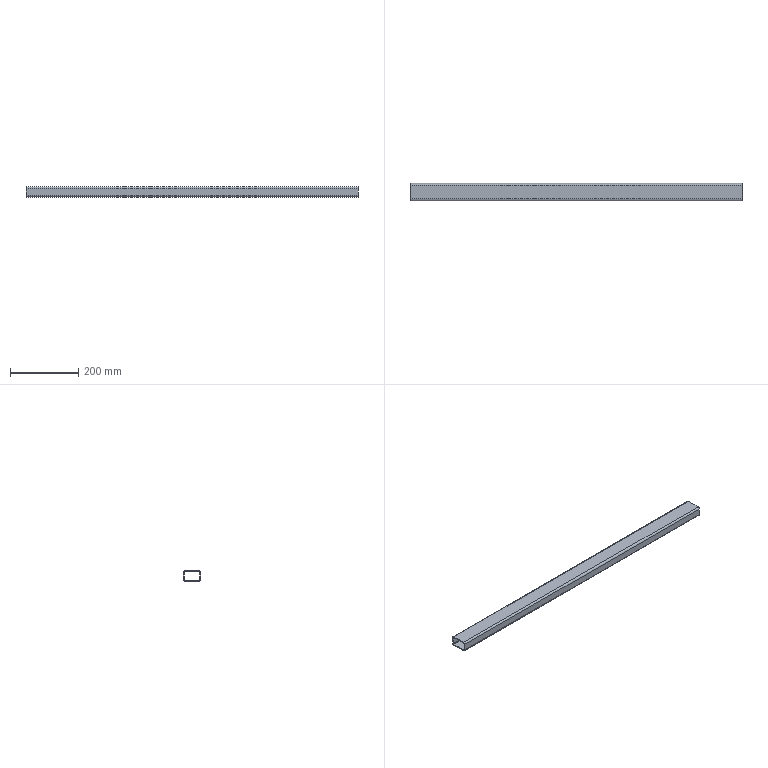Component | SolidWorks | Frame-1_SquareTube10-1 | 1 solid | 18 faces | box 970 x 50 x 30 mm | volume 360405 mm3 | plane 10 | cylinder 8 | commonest cylinder face diameters 5.2 x4 10.4 x4
STEP:
#1=CARTESIAN_POINT('',(19.094,-11.622,-6.402));
#2=VERTEX_POINT('',#1);
#3=CARTESIAN_POINT('',(19.094,-13.181,-6.402));
#4=VERTEX_POINT('',#3);
#5=CARTESIAN_POINT('',(19.094,-11.622,-6.402));
#6=DIRECTION('',(0.,-1.,0.));
#7=VECTOR('',#6,39.37);
#8=LINE('',#5,#7);
#9=EDGE_CURVE('',#2,#4,#8,.T.);
#10=ORIENTED_EDGE('',*,*,#9,.T.);
#11=CARTESIAN_POINT('',(-19.094,-13.181,-6.402));
#12=VERTEX_POINT('',#11);
#13=CARTESIAN_POINT('',(-19.685,-13.181,-6.402));
#14=DIRECTION('',(-1.,0.,0.));
#15=VECTOR('',#14,39.37);
#16=LINE('',#13,#15);
#17=EDGE_CURVE('',#4,#12,#16,.T.);
#18=ORIENTED_EDGE('',*,*,#17,.T.);
#19=CARTESIAN_POINT('',(-19.094,-11.622,-6.402));
#20=VERTEX_POINT('',#19);
#21=CARTESIAN_POINT('',(-19.094,-11.622,-6.402));
#22=DIRECTION('',(0.,1.,0.));
#23=VECTOR('',#22,39.37);
#24=LINE('',#21,#23);
#25=EDGE_CURVE('',#12,#20,#24,.T.);
#26=ORIENTED_EDGE('',*,*,#25,.T.);
#27=CARTESIAN_POINT('',(-19.685,-11.622,-6.402));
#28=DIRECTION('',(1.,0.,0.));
#29=VECTOR('',#28,39.37);
#30=LINE('',#27,#29);
#31=EDGE_CURVE('',#20,#2,#30,.T.);
#32=ORIENTED_EDGE('',*,*,#31,.T.);
#33=EDGE_LOOP('',(#10,#18,#26,#32));
#34=FACE_OUTER_BOUND('',#33,.T.);
#35=CARTESIAN_POINT('',(-19.685,-11.622,-6.402));
#36=DIRECTION('',(0.,0.,-1.));
#37=DIRECTION('',(-1.,0.,0.));
#38=AXIS2_PLACEMENT_3D('',#35,#36,#37);
#39=PLANE('',#38);
#40=ADVANCED_FACE('',(#34),#39,.T.);
#41=ORIENTED_EDGE('',*,*,#17,.F.);
#42=CARTESIAN_POINT('',(19.094,-13.283,-6.504));
#43=VERTEX_POINT('',#42);
#44=CARTESIAN_POINT('',(19.094,-13.181,-6.504));
#45=DIRECTION('',(-1.,0.,0.));
#46=DIRECTION('',(0.,0.,-1.));
#47=AXIS2_PLACEMENT_3D('',#44,#45,#46);
#48=CIRCLE('',#47,0.1024);
#49=EDGE_CURVE('',#43,#4,#48,.T.);
#50=ORIENTED_EDGE('',*,*,#49,.F.);
#51=CARTESIAN_POINT('',(-19.094,-13.283,-6.504));
#52=VERTEX_POINT('',#51);
#53=CARTESIAN_POINT('',(-19.685,-13.283,-6.504));
#54=DIRECTION('',(1.,0.,0.));
#55=VECTOR('',#54,39.37);
#56=LINE('',#53,#55);
#57=EDGE_CURVE('',#52,#43,#56,.T.);
#58=ORIENTED_EDGE('',*,*,#57,.F.);
#59=CARTESIAN_POINT('',(-19.094,-13.181,-6.504));
#60=DIRECTION('',(1.,0.,0.));
#61=DIRECTION('',(0.,0.,-1.));
#62=AXIS2_PLACEMENT_3D('',#59,#60,#61);
#63=CIRCLE('',#62,0.1024);
#64=EDGE_CURVE('',#12,#52,#63,.T.);
#65=ORIENTED_EDGE('',*,*,#64,.F.);
#66=EDGE_LOOP('',(#41,#50,#58,#65));
#67=FACE_OUTER_BOUND('',#66,.T.);
#68=CARTESIAN_POINT('',(-19.685,-13.181,-6.504));
#69=DIRECTION('',(1.,0.,0.));
#70=DIRECTION('',(0.,0.,-1.));
#71=AXIS2_PLACEMENT_3D('',#68,#69,#70);
#72=CYLINDRICAL_SURFACE('',#71,0.1024);
#73=ADVANCED_FACE('',(#67),#72,.F.);
#74=CARTESIAN_POINT('',(19.094,-13.386,-6.504));
#75=VERTEX_POINT('',#74);
#76=CARTESIAN_POINT('',(19.094,-13.181,-6.299));
#77=VERTEX_POINT('',#76);
#78=CARTESIAN_POINT('',(19.094,-13.181,-6.504));
#79=DIRECTION('',(-1.,0.,0.));
#80=DIRECTION('',(0.,0.,-1.));
#81=AXIS2_PLACEMENT_3D('',#78,#79,#80);
#82=CIRCLE('',#81,0.2047);
#83=EDGE_CURVE('',#75,#77,#82,.T.);
#84=ORIENTED_EDGE('',*,*,#83,.F.);
#85=CARTESIAN_POINT('',(19.094,-13.386,-7.276));
#86=VERTEX_POINT('',#85);
#87=CARTESIAN_POINT('',(19.094,-13.386,6.496));
#88=DIRECTION('',(0.,0.,1.));
#89=VECTOR('',#88,39.37);
#90=LINE('',#87,#89);
#91=EDGE_CURVE('',#86,#75,#90,.T.);
#92=ORIENTED_EDGE('',*,*,#91,.F.);
#93=CARTESIAN_POINT('',(19.094,-13.181,-7.48));
#94=VERTEX_POINT('',#93);
#95=CARTESIAN_POINT('',(19.094,-13.181,-7.276));
#96=DIRECTION('',(-1.,0.,0.));
#97=DIRECTION('',(0.,0.,-1.));
#98=AXIS2_PLACEMENT_3D('',#95,#96,#97);
#99=CIRCLE('',#98,0.2047);
#100=EDGE_CURVE('',#94,#86,#99,.T.);
#101=ORIENTED_EDGE('',*,*,#100,.F.);
#102=CARTESIAN_POINT('',(19.094,-11.622,-7.48));
#103=VERTEX_POINT('',#102);
#104=CARTESIAN_POINT('',(19.094,-10.335,-7.48));
#105=DIRECTION('',(0.,-1.,0.));
#106=VECTOR('',#105,39.37);
#107=LINE('',#104,#106);
#108=EDGE_CURVE('',#103,#94,#107,.T.);
#109=ORIENTED_EDGE('',*,*,#108,.F.);
#110=CARTESIAN_POINT('',(19.094,-11.417,-7.276));
#111=VERTEX_POINT('',#110);
#112=CARTESIAN_POINT('',(19.094,-11.622,-7.276));
#113=DIRECTION('',(-1.,0.,0.));
#114=DIRECTION('',(0.,0.,-1.));
#115=AXIS2_PLACEMENT_3D('',#112,#113,#114);
#116=CIRCLE('',#115,0.2047);
#117=EDGE_CURVE('',#111,#103,#116,.T.);
#118=ORIENTED_EDGE('',*,*,#117,.F.);
#119=CARTESIAN_POINT('',(19.094,-11.417,-6.504));
#120=VERTEX_POINT('',#119);
#121=CARTESIAN_POINT('',(19.094,-11.417,6.496));
#122=DIRECTION('',(0.,0.,-1.));
#123=VECTOR('',#122,39.37);
#124=LINE('',#121,#123);
#125=EDGE_CURVE('',#120,#111,#124,.T.);
#126=ORIENTED_EDGE('',*,*,#125,.F.);
#127=CARTESIAN_POINT('',(19.094,-11.622,-6.299));
#128=VERTEX_POINT('',#127);
#129=CARTESIAN_POINT('',(19.094,-11.622,-6.504));
#130=DIRECTION('',(-1.,0.,0.));
#131=DIRECTION('',(0.,0.,-1.));
#132=AXIS2_PLACEMENT_3D('',#129,#130,#131);
#133=CIRCLE('',#132,0.2047);
#134=EDGE_CURVE('',#128,#120,#133,.T.);
#135=ORIENTED_EDGE('',*,*,#134,.F.);
#136=CARTESIAN_POINT('',(19.094,-10.335,-6.299));
#137=DIRECTION('',(0.,1.,0.));
#138=VECTOR('',#137,39.37);
#139=LINE('',#136,#138);
#140=EDGE_CURVE('',#77,#128,#139,.T.);
#141=ORIENTED_EDGE('',*,*,#140,.F.);
#142=EDGE_LOOP('',(#84,#92,#101,#109,#118,#126,#135,#141));
#143=FACE_OUTER_BOUND('',#142,.T.);
#144=CARTESIAN_POINT('',(19.094,-13.181,-7.378));
#145=VERTEX_POINT('',#144);
#146=CARTESIAN_POINT('',(19.094,-11.622,-7.378));
#147=VERTEX_POINT('',#146);
#148=CARTESIAN_POINT('',(19.094,-10.335,-7.378));
#149=DIRECTION('',(0.,1.,0.));
#150=VECTOR('',#149,39.37);
#151=LINE('',#148,#150);
#152=EDGE_CURVE('',#145,#147,#151,.T.);
#153=ORIENTED_EDGE('',*,*,#152,.F.);
#154=CARTESIAN_POINT('',(19.094,-13.283,-7.276));
#155=VERTEX_POINT('',#154);
#156=CARTESIAN_POINT('',(19.094,-13.181,-7.276));
#157=DIRECTION('',(1.,0.,0.));
#158=DIRECTION('',(0.,0.,-1.));
#159=AXIS2_PLACEMENT_3D('',#156,#157,#158);
#160=CIRCLE('',#159,0.1024);
#161=EDGE_CURVE('',#155,#145,#160,.T.);
#162=ORIENTED_EDGE('',*,*,#161,.F.);
#163=CARTESIAN_POINT('',(19.094,-13.283,6.496));
#164=DIRECTION('',(0.,0.,-1.));
#165=VECTOR('',#164,39.37);
#166=LINE('',#163,#165);
#167=EDGE_CURVE('',#43,#155,#166,.T.);
#168=ORIENTED_EDGE('',*,*,#167,.F.);
#169=ORIENTED_EDGE('',*,*,#49,.T.);
#170=ORIENTED_EDGE('',*,*,#9,.F.);
#171=CARTESIAN_POINT('',(19.094,-11.52,-6.504));
#172=VERTEX_POINT('',#171);
#173=CARTESIAN_POINT('',(19.094,-11.622,-6.504));
#174=DIRECTION('',(1.,0.,0.));
#175=DIRECTION('',(0.,0.,-1.));
#176=AXIS2_PLACEMENT_3D('',#173,#174,#175);
#177=CIRCLE('',#176,0.1024);
#178=EDGE_CURVE('',#172,#2,#177,.T.);
#179=ORIENTED_EDGE('',*,*,#178,.F.);
#180=CARTESIAN_POINT('',(19.094,-11.52,-7.276));
#181=VERTEX_POINT('',#180);
#182=CARTESIAN_POINT('',(19.094,-11.52,6.496));
#183=DIRECTION('',(0.,0.,1.));
#184=VECTOR('',#183,39.37);
#185=LINE('',#182,#184);
#186=EDGE_CURVE('',#181,#172,#185,.T.);
#187=ORIENTED_EDGE('',*,*,#186,.F.);
#188=CARTESIAN_POINT('',(19.094,-11.622,-7.276));
#189=DIRECTION('',(1.,0.,0.));
#190=DIRECTION('',(0.,0.,-1.));
#191=AXIS2_PLACEMENT_3D('',#188,#189,#190);
#192=CIRCLE('',#191,0.1024);
#193=EDGE_CURVE('',#147,#181,#192,.T.);
#194=ORIENTED_EDGE('',*,*,#193,.F.);
#195=EDGE_LOOP('',(#153,#162,#168,#169,#170,#179,#187,#194));
#196=FACE_BOUND('',#195,.T.);
#197=CARTESIAN_POINT('',(19.094,-10.335,6.496));
#198=DIRECTION('',(-1.,0.,0.));
#199=DIRECTION('',(0.,0.,1.));
#200=AXIS2_PLACEMENT_3D('',#197,#198,#199);
#201=PLANE('',#200);
#202=ADVANCED_FACE('',(#143,#196),#201,.F.);
#203=CARTESIAN_POINT('',(-19.094,-11.52,-6.504));
#204=VERTEX_POINT('',#203);
#205=CARTESIAN_POINT('',(-19.685,-11.52,-6.504));
#206=DIRECTION('',(-1.,0.,0.));
#207=VECTOR('',#206,39.37);
#208=LINE('',#205,#207);
#209=EDGE_CURVE('',#172,#204,#208,.T.);
#210=ORIENTED_EDGE('',*,*,#209,.F.);
#211=ORIENTED_EDGE('',*,*,#178,.T.);
#212=ORIENTED_EDGE('',*,*,#31,.F.);
#213=CARTESIAN_POINT('',(-19.094,-11.622,-6.504));
#214=DIRECTION('',(1.,0.,0.));
#215=DIRECTION('',(0.,0.,-1.));
#216=AXIS2_PLACEMENT_3D('',#213,#214,#215);
#217=CIRCLE('',#216,0.1024);
#218=EDGE_CURVE('',#204,#20,#217,.T.);
#219=ORIENTED_EDGE('',*,*,#218,.F.);
#220=EDGE_LOOP('',(#210,#211,#212,#219));
#221=FACE_OUTER_BOUND('',#220,.T.);
#222=CARTESIAN_POINT('',(-19.685,-11.622,-6.504));
#223=DIRECTION('',(1.,0.,0.));
#224=DIRECTION('',(0.,0.,-1.));
#225=AXIS2_PLACEMENT_3D('',#222,#223,#224);
#226=CYLINDRICAL_SURFACE('',#225,0.1024);
#227=ADVANCED_FACE('',(#221),#226,.F.);
#228=CARTESIAN_POINT('',(-19.094,-11.417,-6.504));
#229=VERTEX_POINT('',#228);
#230=CARTESIAN_POINT('',(-19.094,-11.622,-6.299));
#231=VERTEX_POINT('',#230);
#232=CARTESIAN_POINT('',(-19.094,-11.622,-6.504));
#233=DIRECTION('',(1.,0.,0.));
#234=DIRECTION('',(0.,0.,-1.));
#235=AXIS2_PLACEMENT_3D('',#232,#233,#234);
#236=CIRCLE('',#235,0.2047);
#237=EDGE_CURVE('',#229,#231,#236,.T.);
#238=ORIENTED_EDGE('',*,*,#237,.F.);
#239=CARTESIAN_POINT('',(-19.094,-11.417,-7.276));
#240=VERTEX_POINT('',#239);
#241=CARTESIAN_POINT('',(-19.094,-11.417,6.496));
#242=DIRECTION('',(0.,0.,1.));
#243=VECTOR('',#242,39.37);
#244=LINE('',#241,#243);
#245=EDGE_CURVE('',#240,#229,#244,.T.);
#246=ORIENTED_EDGE('',*,*,#245,.F.);
#247=CARTESIAN_POINT('',(-19.094,-11.622,-7.48));
#248=VERTEX_POINT('',#247);
#249=CARTESIAN_POINT('',(-19.094,-11.622,-7.276));
#250=DIRECTION('',(1.,0.,0.));
#251=DIRECTION('',(0.,0.,-1.));
#252=AXIS2_PLACEMENT_3D('',#249,#250,#251);
#253=CIRCLE('',#252,0.2047);
#254=EDGE_CURVE('',#248,#240,#253,.T.);
#255=ORIENTED_EDGE('',*,*,#254,.F.);
#256=CARTESIAN_POINT('',(-19.094,-13.181,-7.48));
#257=VERTEX_POINT('',#256);
#258=CARTESIAN_POINT('',(-19.094,-10.335,-7.48));
#259=DIRECTION('',(0.,1.,0.));
#260=VECTOR('',#259,39.37);
#261=LINE('',#258,#260);
#262=EDGE_CURVE('',#257,#248,#261,.T.);
#263=ORIENTED_EDGE('',*,*,#262,.F.);
#264=CARTESIAN_POINT('',(-19.094,-13.386,-7.276));
#265=VERTEX_POINT('',#264);
#266=CARTESIAN_POINT('',(-19.094,-13.181,-7.276));
#267=DIRECTION('',(1.,0.,0.));
#268=DIRECTION('',(0.,0.,-1.));
#269=AXIS2_PLACEMENT_3D('',#266,#267,#268);
#270=CIRCLE('',#269,0.2047);
#271=EDGE_CURVE('',#265,#257,#270,.T.);
#272=ORIENTED_EDGE('',*,*,#271,.F.);
#273=CARTESIAN_POINT('',(-19.094,-13.386,-6.504));
#274=VERTEX_POINT('',#273);
#275=CARTESIAN_POINT('',(-19.094,-13.386,6.496));
#276=DIRECTION('',(0.,0.,-1.));
#277=VECTOR('',#276,39.37);
#278=LINE('',#275,#277);
#279=EDGE_CURVE('',#274,#265,#278,.T.);
#280=ORIENTED_EDGE('',*,*,#279,.F.);
#281=CARTESIAN_POINT('',(-19.094,-13.181,-6.299));
#282=VERTEX_POINT('',#281);
#283=CARTESIAN_POINT('',(-19.094,-13.181,-6.504));
#284=DIRECTION('',(1.,0.,0.));
#285=DIRECTION('',(0.,0.,-1.));
#286=AXIS2_PLACEMENT_3D('',#283,#284,#285);
#287=CIRCLE('',#286,0.2047);
#288=EDGE_CURVE('',#282,#274,#287,.T.);
#289=ORIENTED_EDGE('',*,*,#288,.F.);
#290=CARTESIAN_POINT('',(-19.094,-10.335,-6.299));
#291=DIRECTION('',(0.,-1.,0.));
#292=VECTOR('',#291,39.37);
#293=LINE('',#290,#292);
#294=EDGE_CURVE('',#231,#282,#293,.T.);
#295=ORIENTED_EDGE('',*,*,#294,.F.);
#296=EDGE_LOOP('',(#238,#246,#255,#263,#272,#280,#289,#295));
#297=FACE_OUTER_BOUND('',#296,.T.);
#298=CARTESIAN_POINT('',(-19.094,-11.52,-7.276));
#299=VERTEX_POINT('',#298);
#300=CARTESIAN_POINT('',(-19.094,-11.622,-7.378));
#301=VERTEX_POINT('',#300);
#302=CARTESIAN_POINT('',(-19.094,-11.622,-7.276));
#303=DIRECTION('',(-1.,0.,0.));
#304=DIRECTION('',(0.,0.,-1.));
#305=AXIS2_PLACEMENT_3D('',#302,#303,#304);
#306=CIRCLE('',#305,0.1024);
#307=EDGE_CURVE('',#299,#301,#306,.T.);
#308=ORIENTED_EDGE('',*,*,#307,.F.);
#309=CARTESIAN_POINT('',(-19.094,-11.52,6.496));
#310=DIRECTION('',(0.,0.,-1.));
#311=VECTOR('',#310,39.37);
#312=LINE('',#309,#311);
#313=EDGE_CURVE('',#204,#299,#312,.T.);
#314=ORIENTED_EDGE('',*,*,#313,.F.);
#315=ORIENTED_EDGE('',*,*,#218,.T.);
#316=ORIENTED_EDGE('',*,*,#25,.F.);
#317=ORIENTED_EDGE('',*,*,#64,.T.);
#318=CARTESIAN_POINT('',(-19.094,-13.283,-7.276));
#319=VERTEX_POINT('',#318);
#320=CARTESIAN_POINT('',(-19.094,-13.283,6.496));
#321=DIRECTION('',(0.,0.,1.));
#322=VECTOR('',#321,39.37);
#323=LINE('',#320,#322);
#324=EDGE_CURVE('',#319,#52,#323,.T.);
#325=ORIENTED_EDGE('',*,*,#324,.F.);
#326=CARTESIAN_POINT('',(-19.094,-13.181,-7.378));
#327=VERTEX_POINT('',#326);
#328=CARTESIAN_POINT('',(-19.094,-13.181,-7.276));
#329=DIRECTION('',(-1.,0.,0.));
#330=DIRECTION('',(0.,0.,-1.));
#331=AXIS2_PLACEMENT_3D('',#328,#329,#330);
#332=CIRCLE('',#331,0.1024);
#333=EDGE_CURVE('',#327,#319,#332,.T.);
#334=ORIENTED_EDGE('',*,*,#333,.F.);
#335=CARTESIAN_POINT('',(-19.094,-10.335,-7.378));
#336=DIRECTION('',(0.,-1.,0.));
#337=VECTOR('',#336,39.37);
#338=LINE('',#335,#337);
#339=EDGE_CURVE('',#301,#327,#338,.T.);
#340=ORIENTED_EDGE('',*,*,#339,.F.);
#341=EDGE_LOOP('',(#308,#314,#315,#316,#317,#325,#334,#340));
#342=FACE_BOUND('',#341,.T.);
#343=CARTESIAN_POINT('',(-19.094,-10.335,6.496));
#344=DIRECTION('',(1.,0.,0.));
#345=DIRECTION('',(0.,0.,-1.));
#346=AXIS2_PLACEMENT_3D('',#343,#344,#345);
#347=PLANE('',#346);
#348=ADVANCED_FACE('',(#297,#342),#347,.F.);
#349=ORIENTED_EDGE('',*,*,#167,.T.);
#350=CARTESIAN_POINT('',(-19.685,-13.283,-7.276));
#351=DIRECTION('',(-1.,0.,0.));
#352=VECTOR('',#351,39.37);
#353=LINE('',#350,#352);
#354=EDGE_CURVE('',#155,#319,#353,.T.);
#355=ORIENTED_EDGE('',*,*,#354,.T.);
#356=ORIENTED_EDGE('',*,*,#324,.T.);
#357=ORIENTED_EDGE('',*,*,#57,.T.);
#358=EDGE_LOOP('',(#349,#355,#356,#357));
#359=FACE_OUTER_BOUND('',#358,.T.);
#360=CARTESIAN_POINT('',(-19.685,-13.283,-7.276));
#361=DIRECTION('',(0.,1.,0.));
#362=DIRECTION('',(0.,0.,1.));
#363=AXIS2_PLACEMENT_3D('',#360,#361,#362);
#364=PLANE('',#363);
#365=ADVANCED_FACE('',(#359),#364,.T.);
#366=ORIENTED_EDGE('',*,*,#294,.T.);
#367=CARTESIAN_POINT('',(-19.685,-13.181,-6.299));
#368=DIRECTION('',(-1.,0.,0.));
#369=VECTOR('',#368,39.37);
#370=LINE('',#367,#369);
#371=EDGE_CURVE('',#77,#282,#370,.T.);
#372=ORIENTED_EDGE('',*,*,#371,.F.);
#373=ORIENTED_EDGE('',*,*,#140,.T.);
#374=CARTESIAN_POINT('',(-19.685,-11.622,-6.299));
#375=DIRECTION('',(1.,0.,0.));
#376=VECTOR('',#375,39.37);
#377=LINE('',#374,#376);
#378=EDGE_CURVE('',#231,#128,#377,.T.);
#379=ORIENTED_EDGE('',*,*,#378,.F.);
#380=EDGE_LOOP('',(#366,#372,#373,#379));
#381=FACE_OUTER_BOUND('',#380,.T.);
#382=CARTESIAN_POINT('',(-19.685,-11.622,-6.299));
#383=DIRECTION('',(0.,0.,-1.));
#384=DIRECTION('',(-1.,0.,0.));
#385=AXIS2_PLACEMENT_3D('',#382,#383,#384);
#386=PLANE('',#385);
#387=ADVANCED_FACE('',(#381),#386,.F.);
#388=CARTESIAN_POINT('',(-19.685,-13.386,-6.504));
#389=DIRECTION('',(1.,0.,0.));
#390=VECTOR('',#389,39.37);
#391=LINE('',#388,#390);
#392=EDGE_CURVE('',#274,#75,#391,.T.);
#393=ORIENTED_EDGE('',*,*,#392,.T.);
#394=ORIENTED_EDGE('',*,*,#83,.T.);
#395=ORIENTED_EDGE('',*,*,#371,.T.);
#396=ORIENTED_EDGE('',*,*,#288,.T.);
#397=EDGE_LOOP('',(#393,#394,#395,#396));
#398=FACE_OUTER_BOUND('',#397,.T.);
#399=CARTESIAN_POINT('',(-19.685,-13.181,-6.504));
#400=DIRECTION('',(1.,0.,0.));
#401=DIRECTION('',(0.,0.,-1.));
#402=AXIS2_PLACEMENT_3D('',#399,#400,#401);
#403=CYLINDRICAL_SURFACE('',#402,0.2047);
#404=ADVANCED_FACE('',(#398),#403,.T.);
#405=ORIENTED_EDGE('',*,*,#279,.T.);
#406=CARTESIAN_POINT('',(-19.685,-13.386,-7.276));
#407=DIRECTION('',(-1.,0.,0.));
#408=VECTOR('',#407,39.37);
#409=LINE('',#406,#408);
#410=EDGE_CURVE('',#86,#265,#409,.T.);
#411=ORIENTED_EDGE('',*,*,#410,.F.);
#412=ORIENTED_EDGE('',*,*,#91,.T.);
#413=ORIENTED_EDGE('',*,*,#392,.F.);
#414=EDGE_LOOP('',(#405,#411,#412,#413));
#415=FACE_OUTER_BOUND('',#414,.T.);
#416=CARTESIAN_POINT('',(-19.685,-13.386,-7.276));
#417=DIRECTION('',(0.,1.,0.));
#418=DIRECTION('',(0.,0.,1.));
#419=AXIS2_PLACEMENT_3D('',#416,#417,#418);
#420=PLANE('',#419);
#421=ADVANCED_FACE('',(#415),#420,.F.);
#422=CARTESIAN_POINT('',(-19.685,-13.181,-7.48));
#423=DIRECTION('',(1.,0.,0.));
#424=VECTOR('',#423,39.37);
#425=LINE('',#422,#424);
#426=EDGE_CURVE('',#257,#94,#425,.T.);
#427=ORIENTED_EDGE('',*,*,#426,.T.);
#428=ORIENTED_EDGE('',*,*,#100,.T.);
#429=ORIENTED_EDGE('',*,*,#410,.T.);
#430=ORIENTED_EDGE('',*,*,#271,.T.);
#431=EDGE_LOOP('',(#427,#428,#429,#430));
#432=FACE_OUTER_BOUND('',#431,.T.);
#433=CARTESIAN_POINT('',(-19.685,-13.181,-7.276));
#434=DIRECTION('',(1.,0.,0.));
#435=DIRECTION('',(0.,0.,-1.));
#436=AXIS2_PLACEMENT_3D('',#433,#434,#435);
#437=CYLINDRICAL_SURFACE('',#436,0.2047);
#438=ADVANCED_FACE('',(#432),#437,.T.);
#439=ORIENTED_EDGE('',*,*,#262,.T.);
#440=CARTESIAN_POINT('',(-19.685,-11.622,-7.48));
#441=DIRECTION('',(-1.,0.,0.));
#442=VECTOR('',#441,39.37);
#443=LINE('',#440,#442);
#444=EDGE_CURVE('',#103,#248,#443,.T.);
#445=ORIENTED_EDGE('',*,*,#444,.F.);
#446=ORIENTED_EDGE('',*,*,#108,.T.);
#447=ORIENTED_EDGE('',*,*,#426,.F.);
#448=EDGE_LOOP('',(#439,#445,#446,#447));
#449=FACE_OUTER_BOUND('',#448,.T.);
#450=CARTESIAN_POINT('',(-19.685,-13.181,-7.48));
#451=DIRECTION('',(0.,0.,1.));
#452=DIRECTION('',(1.,0.,0.));
#453=AXIS2_PLACEMENT_3D('',#450,#451,#452);
#454=PLANE('',#453);
#455=ADVANCED_FACE('',(#449),#454,.F.);
#456=CARTESIAN_POINT('',(-19.685,-11.417,-7.276));
#457=DIRECTION('',(1.,0.,0.));
#458=VECTOR('',#457,39.37);
#459=LINE('',#456,#458);
#460=EDGE_CURVE('',#240,#111,#459,.T.);
#461=ORIENTED_EDGE('',*,*,#460,.T.);
#462=ORIENTED_EDGE('',*,*,#117,.T.);
#463=ORIENTED_EDGE('',*,*,#444,.T.);
#464=ORIENTED_EDGE('',*,*,#254,.T.);
#465=EDGE_LOOP('',(#461,#462,#463,#464));
#466=FACE_OUTER_BOUND('',#465,.T.);
#467=CARTESIAN_POINT('',(-19.685,-11.622,-7.276));
#468=DIRECTION('',(1.,0.,0.));
#469=DIRECTION('',(0.,0.,-1.));
#470=AXIS2_PLACEMENT_3D('',#467,#468,#469);
#471=CYLINDRICAL_SURFACE('',#470,0.2047);
#472=ADVANCED_FACE('',(#466),#471,.T.);
#473=ORIENTED_EDGE('',*,*,#245,.T.);
#474=CARTESIAN_POINT('',(-19.685,-11.417,-6.504));
#475=DIRECTION('',(-1.,0.,0.));
#476=VECTOR('',#475,39.37);
#477=LINE('',#474,#476);
#478=EDGE_CURVE('',#120,#229,#477,.T.);
#479=ORIENTED_EDGE('',*,*,#478,.F.);
#480=ORIENTED_EDGE('',*,*,#125,.T.);
#481=ORIENTED_EDGE('',*,*,#460,.F.);
#482=EDGE_LOOP('',(#473,#479,#480,#481));
#483=FACE_OUTER_BOUND('',#482,.T.);
#484=CARTESIAN_POINT('',(-19.685,-11.417,-6.504));
#485=DIRECTION('',(0.,-1.,0.));
#486=DIRECTION('',(0.,0.,-1.));
#487=AXIS2_PLACEMENT_3D('',#484,#485,#486);
#488=PLANE('',#487);
#489=ADVANCED_FACE('',(#483),#488,.F.);
#490=ORIENTED_EDGE('',*,*,#378,.T.);
#491=ORIENTED_EDGE('',*,*,#134,.T.);
#492=ORIENTED_EDGE('',*,*,#478,.T.);
#493=ORIENTED_EDGE('',*,*,#237,.T.);
#494=EDGE_LOOP('',(#490,#491,#492,#493));
#495=FACE_OUTER_BOUND('',#494,.T.);
#496=CARTESIAN_POINT('',(-19.685,-11.622,-6.504));
#497=DIRECTION('',(1.,0.,0.));
#498=DIRECTION('',(0.,0.,-1.));
#499=AXIS2_PLACEMENT_3D('',#496,#497,#498);
#500=CYLINDRICAL_SURFACE('',#499,0.2047);
#501=ADVANCED_FACE('',(#495),#500,.T.);
#502=CARTESIAN_POINT('',(-19.685,-11.622,-7.378));
#503=DIRECTION('',(-1.,0.,0.));
#504=VECTOR('',#503,39.37);
#505=LINE('',#502,#504);
#506=EDGE_CURVE('',#147,#301,#505,.T.);
#507=ORIENTED_EDGE('',*,*,#506,.F.);
#508=ORIENTED_EDGE('',*,*,#193,.T.);
#509=CARTESIAN_POINT('',(-19.685,-11.52,-7.276));
#510=DIRECTION('',(1.,0.,0.));
#511=VECTOR('',#510,39.37);
#512=LINE('',#509,#511);
#513=EDGE_CURVE('',#299,#181,#512,.T.);
#514=ORIENTED_EDGE('',*,*,#513,.F.);
#515=ORIENTED_EDGE('',*,*,#307,.T.);
#516=EDGE_LOOP('',(#507,#508,#514,#515));
#517=FACE_OUTER_BOUND('',#516,.T.);
#518=CARTESIAN_POINT('',(-19.685,-11.622,-7.276));
#519=DIRECTION('',(1.,0.,0.));
#520=DIRECTION('',(0.,0.,-1.));
#521=AXIS2_PLACEMENT_3D('',#518,#519,#520);
#522=CYLINDRICAL_SURFACE('',#521,0.1024);
#523=ADVANCED_FACE('',(#517),#522,.F.);
#524=ORIENTED_EDGE('',*,*,#152,.T.);
#525=ORIENTED_EDGE('',*,*,#506,.T.);
#526=ORIENTED_EDGE('',*,*,#339,.T.);
#527=CARTESIAN_POINT('',(-19.685,-13.181,-7.378));
#528=DIRECTION('',(1.,0.,0.));
#529=VECTOR('',#528,39.37);
#530=LINE('',#527,#529);
#531=EDGE_CURVE('',#327,#145,#530,.T.);
#532=ORIENTED_EDGE('',*,*,#531,.T.);
#533=EDGE_LOOP('',(#524,#525,#526,#532));
#534=FACE_OUTER_BOUND('',#533,.T.);
#535=CARTESIAN_POINT('',(-19.685,-13.181,-7.378));
#536=DIRECTION('',(0.,0.,1.));
#537=DIRECTION('',(1.,0.,0.));
#538=AXIS2_PLACEMENT_3D('',#535,#536,#537);
#539=PLANE('',#538);
#540=ADVANCED_FACE('',(#534),#539,.T.);
#541=ORIENTED_EDGE('',*,*,#354,.F.);
#542=ORIENTED_EDGE('',*,*,#161,.T.);
#543=ORIENTED_EDGE('',*,*,#531,.F.);
#544=ORIENTED_EDGE('',*,*,#333,.T.);
#545=EDGE_LOOP('',(#541,#542,#543,#544));
#546=FACE_OUTER_BOUND('',#545,.T.);
#547=CARTESIAN_POINT('',(-19.685,-13.181,-7.276));
#548=DIRECTION('',(1.,0.,0.));
#549=DIRECTION('',(0.,0.,-1.));
#550=AXIS2_PLACEMENT_3D('',#547,#548,#549);
#551=CYLINDRICAL_SURFACE('',#550,0.1024);
#552=ADVANCED_FACE('',(#546),#551,.F.);
#553=ORIENTED_EDGE('',*,*,#186,.T.);
#554=ORIENTED_EDGE('',*,*,#209,.T.);
#555=ORIENTED_EDGE('',*,*,#313,.T.);
#556=ORIENTED_EDGE('',*,*,#513,.T.);
#557=EDGE_LOOP('',(#553,#554,#555,#556));
#558=FACE_OUTER_BOUND('',#557,.T.);
#559=CARTESIAN_POINT('',(-19.685,-11.52,-6.504));
#560=DIRECTION('',(0.,-1.,0.));
#561=DIRECTION('',(0.,0.,-1.));
#562=AXIS2_PLACEMENT_3D('',#559,#560,#561);
#563=PLANE('',#562);
#564=ADVANCED_FACE('',(#558),#563,.T.);
#565=CLOSED_SHELL('',(#40,#73,#202,#227,#348,#365,#387,#404,#421,#438,#455,#472,#489,#501,#523,#540,#552,#564));
#566=MANIFOLD_SOLID_BREP('',#565);
#567=CARTESIAN_POINT('',(0.,0.,0.));
#568=DIRECTION('',(0.,0.,1.));
#569=DIRECTION('',(1.,0.,0.));
#570=AXIS2_PLACEMENT_3D('',#567,#568,#569);
#571=(LENGTH_UNIT()NAMED_UNIT(*)SI_UNIT($,.METRE.));
#572=LENGTH_MEASURE_WITH_UNIT(LENGTH_MEASURE(0.0254),#571);
#573=DIMENSIONAL_EXPONENTS(1.,0.,0.,0.,0.,0.,0.);
#574=(CONVERSION_BASED_UNIT('',#572)LENGTH_UNIT()NAMED_UNIT(#573));
#575=UNCERTAINTY_MEASURE_WITH_UNIT(LENGTH_MEASURE(0.00001),#574,'','');
#576=(NAMED_UNIT(*)PLANE_ANGLE_UNIT()SI_UNIT($,.RADIAN.));
#577=(NAMED_UNIT(*)SI_UNIT($,.STERADIAN.)SOLID_ANGLE_UNIT());
#578=(GEOMETRIC_REPRESENTATION_CONTEXT(3)GLOBAL_UNCERTAINTY_ASSIGNED_CONTEXT((#575))GLOBAL_UNIT_ASSIGNED_CONTEXT((#574,#576,#577))REPRESENTATION_CONTEXT('',''));
#579=ADVANCED_BREP_SHAPE_REPRESENTATION('',(#566,#570),#578);
#580=COLOUR_RGB('',0.7922,0.8196,0.9333);
#581=FILL_AREA_STYLE_COLOUR('',#580);
#582=FILL_AREA_STYLE('',(#581));
#583=SURFACE_STYLE_FILL_AREA(#582);
#584=SURFACE_SIDE_STYLE('',(#583));
#585=SURFACE_STYLE_USAGE(.BOTH.,#584);
#586=PRESENTATION_STYLE_ASSIGNMENT((#585));
#587=STYLED_ITEM('',(#586),#566);
#588=(LENGTH_UNIT()NAMED_UNIT(*)SI_UNIT($,.METRE.));
#589=LENGTH_MEASURE_WITH_UNIT(LENGTH_MEASURE(0.0254),#588);
#590=DIMENSIONAL_EXPONENTS(1.,0.,0.,0.,0.,0.,0.);
#591=(CONVERSION_BASED_UNIT('',#589)LENGTH_UNIT()NAMED_UNIT(#590));
#592=UNCERTAINTY_MEASURE_WITH_UNIT(LENGTH_MEASURE(0.00001),#591,'','');
#593=(NAMED_UNIT(*)PLANE_ANGLE_UNIT()SI_UNIT($,.RADIAN.));
#594=(NAMED_UNIT(*)SI_UNIT($,.STERADIAN.)SOLID_ANGLE_UNIT());
#595=(GEOMETRIC_REPRESENTATION_CONTEXT(3)GLOBAL_UNCERTAINTY_ASSIGNED_CONTEXT((#592))GLOBAL_UNIT_ASSIGNED_CONTEXT((#591,#593,#594))REPRESENTATION_CONTEXT('',''));
#596=MECHANICAL_DESIGN_GEOMETRIC_PRESENTATION_REPRESENTATION('',(#587),#595);
#597=PRESENTATION_LAYER_ASSIGNMENT('','',(#587));